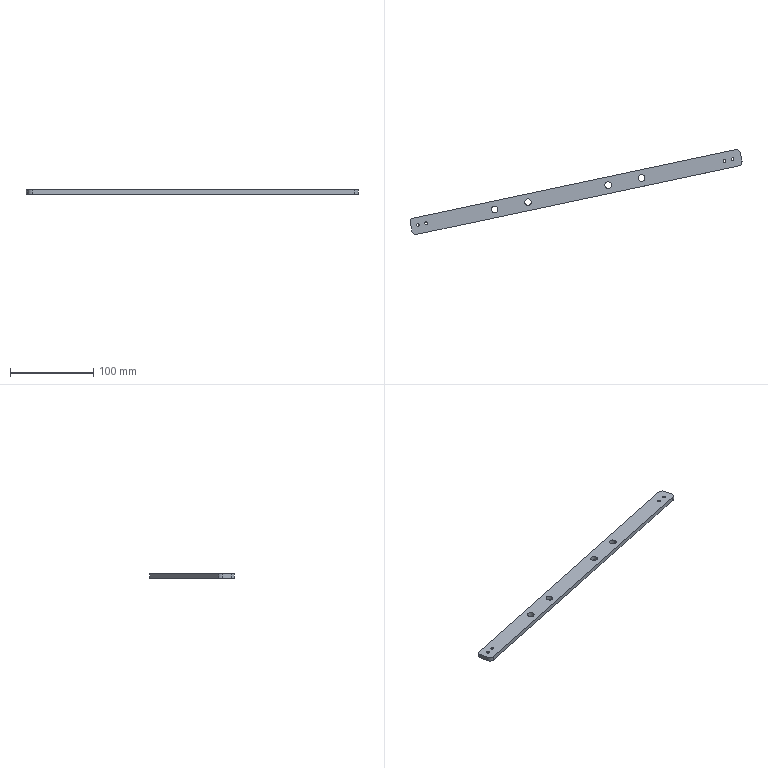Component | SolidWorks | 3UpperBaffle9.26-1 | 1 solid | 26 faces | volume 39132 mm3 | cylinder 20 | plane 6 | commonest cylinder face diameters 3.3 x8 8 x8 10 x4 | material AISI 1045 Steel, Cold Drawn